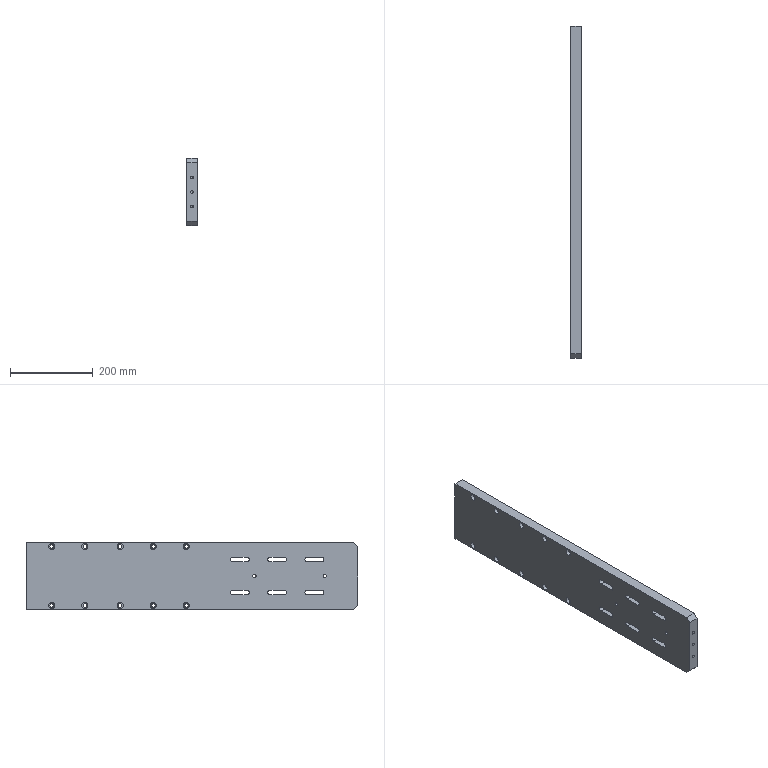Component | SolidWorks | F4-4 | 1 solid | 114 faces | box 25 x 801 x 162 mm | volume 3136886 mm3 | cylinder 70 | plane 30 | cone 14 | commonest cylinder face diameters 15 x20 9 x20 6.8 x14 11 x12 8 x4
build123d program:
from build123d import *

# Parameters (mm, degrees)
SKETCH1_W                                       = 162
SKETCH1_H                                       = 801
BOSS_EXTRUDE1_DEPTH                             = 25
CUT_EXTRUDE1_DEPTH                              = 3570.269
SKETCH12_R                                      = 4
CUT_EXTRUDE2_DEPTH                              = 3570.269
M8_TAPPED_HOLE1_D                               = 6.8
M8_TAPPED_HOLE1_DEPTH                           = 19.75
M8_TAPPED_HOLE1_TIP                             = 2.043
M8_HEX_SOCKET_HEAD_CAP_SCREW_CBORE1_D           = 9
M8_HEX_SOCKET_HEAD_CAP_SCREW_CBORE1_CBORE_D     = 15
M8_HEX_SOCKET_HEAD_CAP_SCREW_CBORE1_CBORE_DEPTH = 8
M8_TAPPED_HOLE2_D                               = 6.8
M8_TAPPED_HOLE2_DEPTH                           = 19.75
M8_TAPPED_HOLE2_TIP                             = 2.043
CHAMFER1_SIZE                                   = 10


with BuildPart() as part:
    # Sketch1 → Boss-Extrude1 (new body)
    with BuildSketch(Plane.XY):
        with Locations((66, 3165.653)):
            Rectangle(SKETCH1_W, SKETCH1_H)
    extrude(amount=BOSS_EXTRUDE1_DEPTH)

    # Sketch11 → Cut-Extrude1 (cut, through all)
    with BuildSketch(Plane.XY.offset(25)):
        with BuildLine():
            Line((100.5, 2852.653), (100.5, 2887.653))
            ThreePointArc((100.5, 2887.653), (106, 2893.153), (111.5, 2887.653))
            Line((111.5, 2887.653), (111.5, 2852.653))
            ThreePointArc((111.5, 2852.653), (106, 2847.153), (100.5, 2852.653))
        make_face()
        with BuildLine():
            Line((20.5, 2852.653), (20.5, 2887.653))
            ThreePointArc((20.5, 2887.653), (26, 2893.153), (31.5, 2887.653))
            Line((31.5, 2887.653), (31.5, 2852.653))
            ThreePointArc((31.5, 2852.653), (26, 2847.153), (20.5, 2852.653))
        make_face()
        with BuildLine():
            Line((100.5, 2942.653), (100.5, 2977.653))
            ThreePointArc((100.5, 2977.653), (106, 2983.153), (111.5, 2977.653))
            Line((111.5, 2977.653), (111.5, 2942.653))
            ThreePointArc((111.5, 2942.653), (106, 2937.153), (100.5, 2942.653))
        make_face()
        with BuildLine():
            Line((20.5, 2942.653), (20.5, 2977.653))
            ThreePointArc((20.5, 2977.653), (26, 2983.153), (31.5, 2977.653))
            Line((31.5, 2977.653), (31.5, 2942.653))
            ThreePointArc((31.5, 2942.653), (26, 2937.153), (20.5, 2942.653))
        make_face()
        with BuildLine():
            Line((100.5, 3032.653), (100.5, 3067.653))
            ThreePointArc((100.5, 3067.653), (106, 3073.153), (111.5, 3067.653))
            Line((111.5, 3067.653), (111.5, 3032.653))
            ThreePointArc((111.5, 3032.653), (106, 3027.153), (100.5, 3032.653))
        make_face()
        with BuildLine():
            Line((20.5, 3032.653), (20.5, 3067.653))
            ThreePointArc((20.5, 3067.653), (26, 3073.153), (31.5, 3067.653))
            Line((31.5, 3067.653), (31.5, 3032.653))
            ThreePointArc((31.5, 3032.653), (26, 3027.153), (20.5, 3032.653))
        make_face()
    extrude(amount=-CUT_EXTRUDE1_DEPTH, mode=Mode.SUBTRACT)

    # Sketch12 → Cut-Extrude2 (cut, through all)
    with BuildSketch(Plane.XY.offset(25)):
        with Locations((66, 2845.153)):
            Circle(SKETCH12_R)
        with Locations((66, 3015.153)):
            Circle(SKETCH12_R)
    extrude(amount=-CUT_EXTRUDE2_DEPTH, mode=Mode.SUBTRACT)

    # M8 Tapped Hole1
    with Locations(Plane.XZ.offset(-2765.153)):
        with Locations((31, 12.5), (66, 12.5), (101, 12.5)):
            Hole(M8_TAPPED_HOLE1_D / 2, depth=M8_TAPPED_HOLE1_DEPTH)
            with Locations((0, 0, -(M8_TAPPED_HOLE1_DEPTH + M8_TAPPED_HOLE1_TIP / 2))):  # 118° drill point
                Cone(0, M8_TAPPED_HOLE1_D / 2, M8_TAPPED_HOLE1_TIP, mode=Mode.SUBTRACT)

    # M8 Hex Socket Head Cap Screw CBORE1 (through all)
    with Locations(Plane(origin=(0, 0, 0), x_dir=(-1, 0, 0), z_dir=(0, 0, -1))):
        with Locations((-137, 3179.153), (-137, 3259.153), (-137, 3339.153), (-137, 3424.153), (-137, 3504.153), (5, 3504.153), (5, 3424.153), (5, 3339.153), (5, 3259.153), (5, 3179.153)):
            CounterBoreHole(M8_HEX_SOCKET_HEAD_CAP_SCREW_CBORE1_D / 2, M8_HEX_SOCKET_HEAD_CAP_SCREW_CBORE1_CBORE_D / 2, M8_HEX_SOCKET_HEAD_CAP_SCREW_CBORE1_CBORE_DEPTH)

    # M8 Tapped Hole2
    with Locations(Plane(origin=(0, 3566.153, 0), x_dir=(-1, 0, 0), z_dir=(0, 1, 0))):
        with Locations((-123.5, 12.5), (-83.5, 12.5), (-48.5, 12.5), (-8.5, 12.5)):
            Hole(M8_TAPPED_HOLE2_D / 2, depth=M8_TAPPED_HOLE2_DEPTH)
            with Locations((0, 0, -(M8_TAPPED_HOLE2_DEPTH + M8_TAPPED_HOLE2_TIP / 2))):  # 118° drill point
                Cone(0, M8_TAPPED_HOLE2_D / 2, M8_TAPPED_HOLE2_TIP, mode=Mode.SUBTRACT)

    # Chamfer1
    chamfer1_edges = [part.edges().sort_by_distance(p)[0] for p in [
        (147, 2765.153, 12.5),
        (-15, 2765.153, 12.5),
    ]]
    chamfer(chamfer1_edges, length=CHAMFER1_SIZE)


solid = part.part

# Placed as in the assembly
solid = solid.moved(Location((96, -2971.874, 10), (0, 90, 0)))